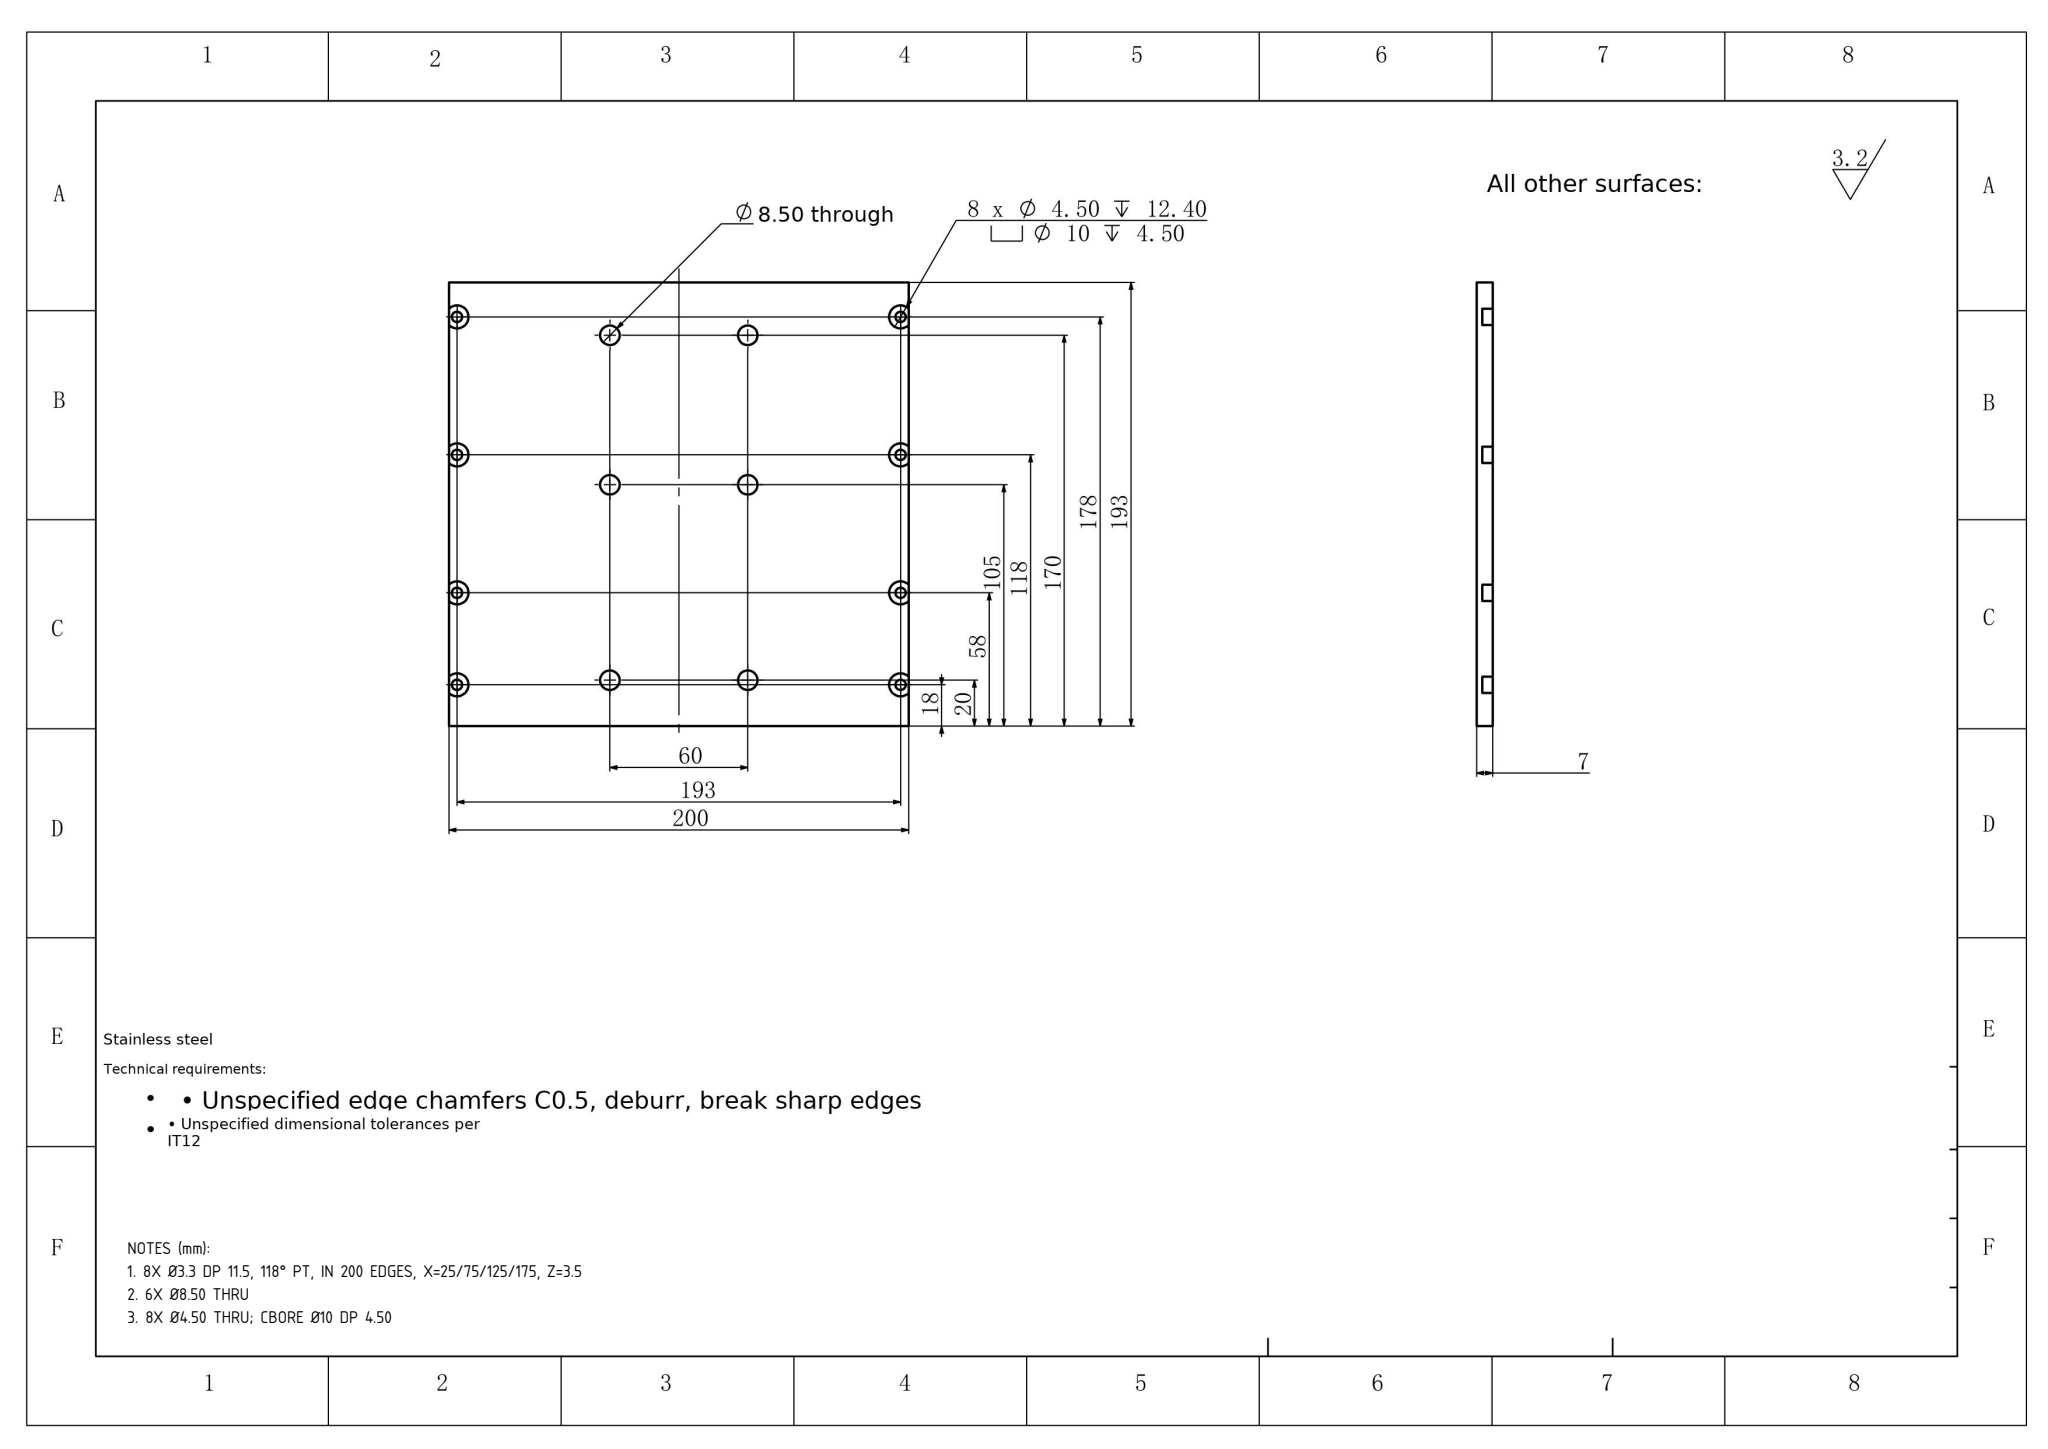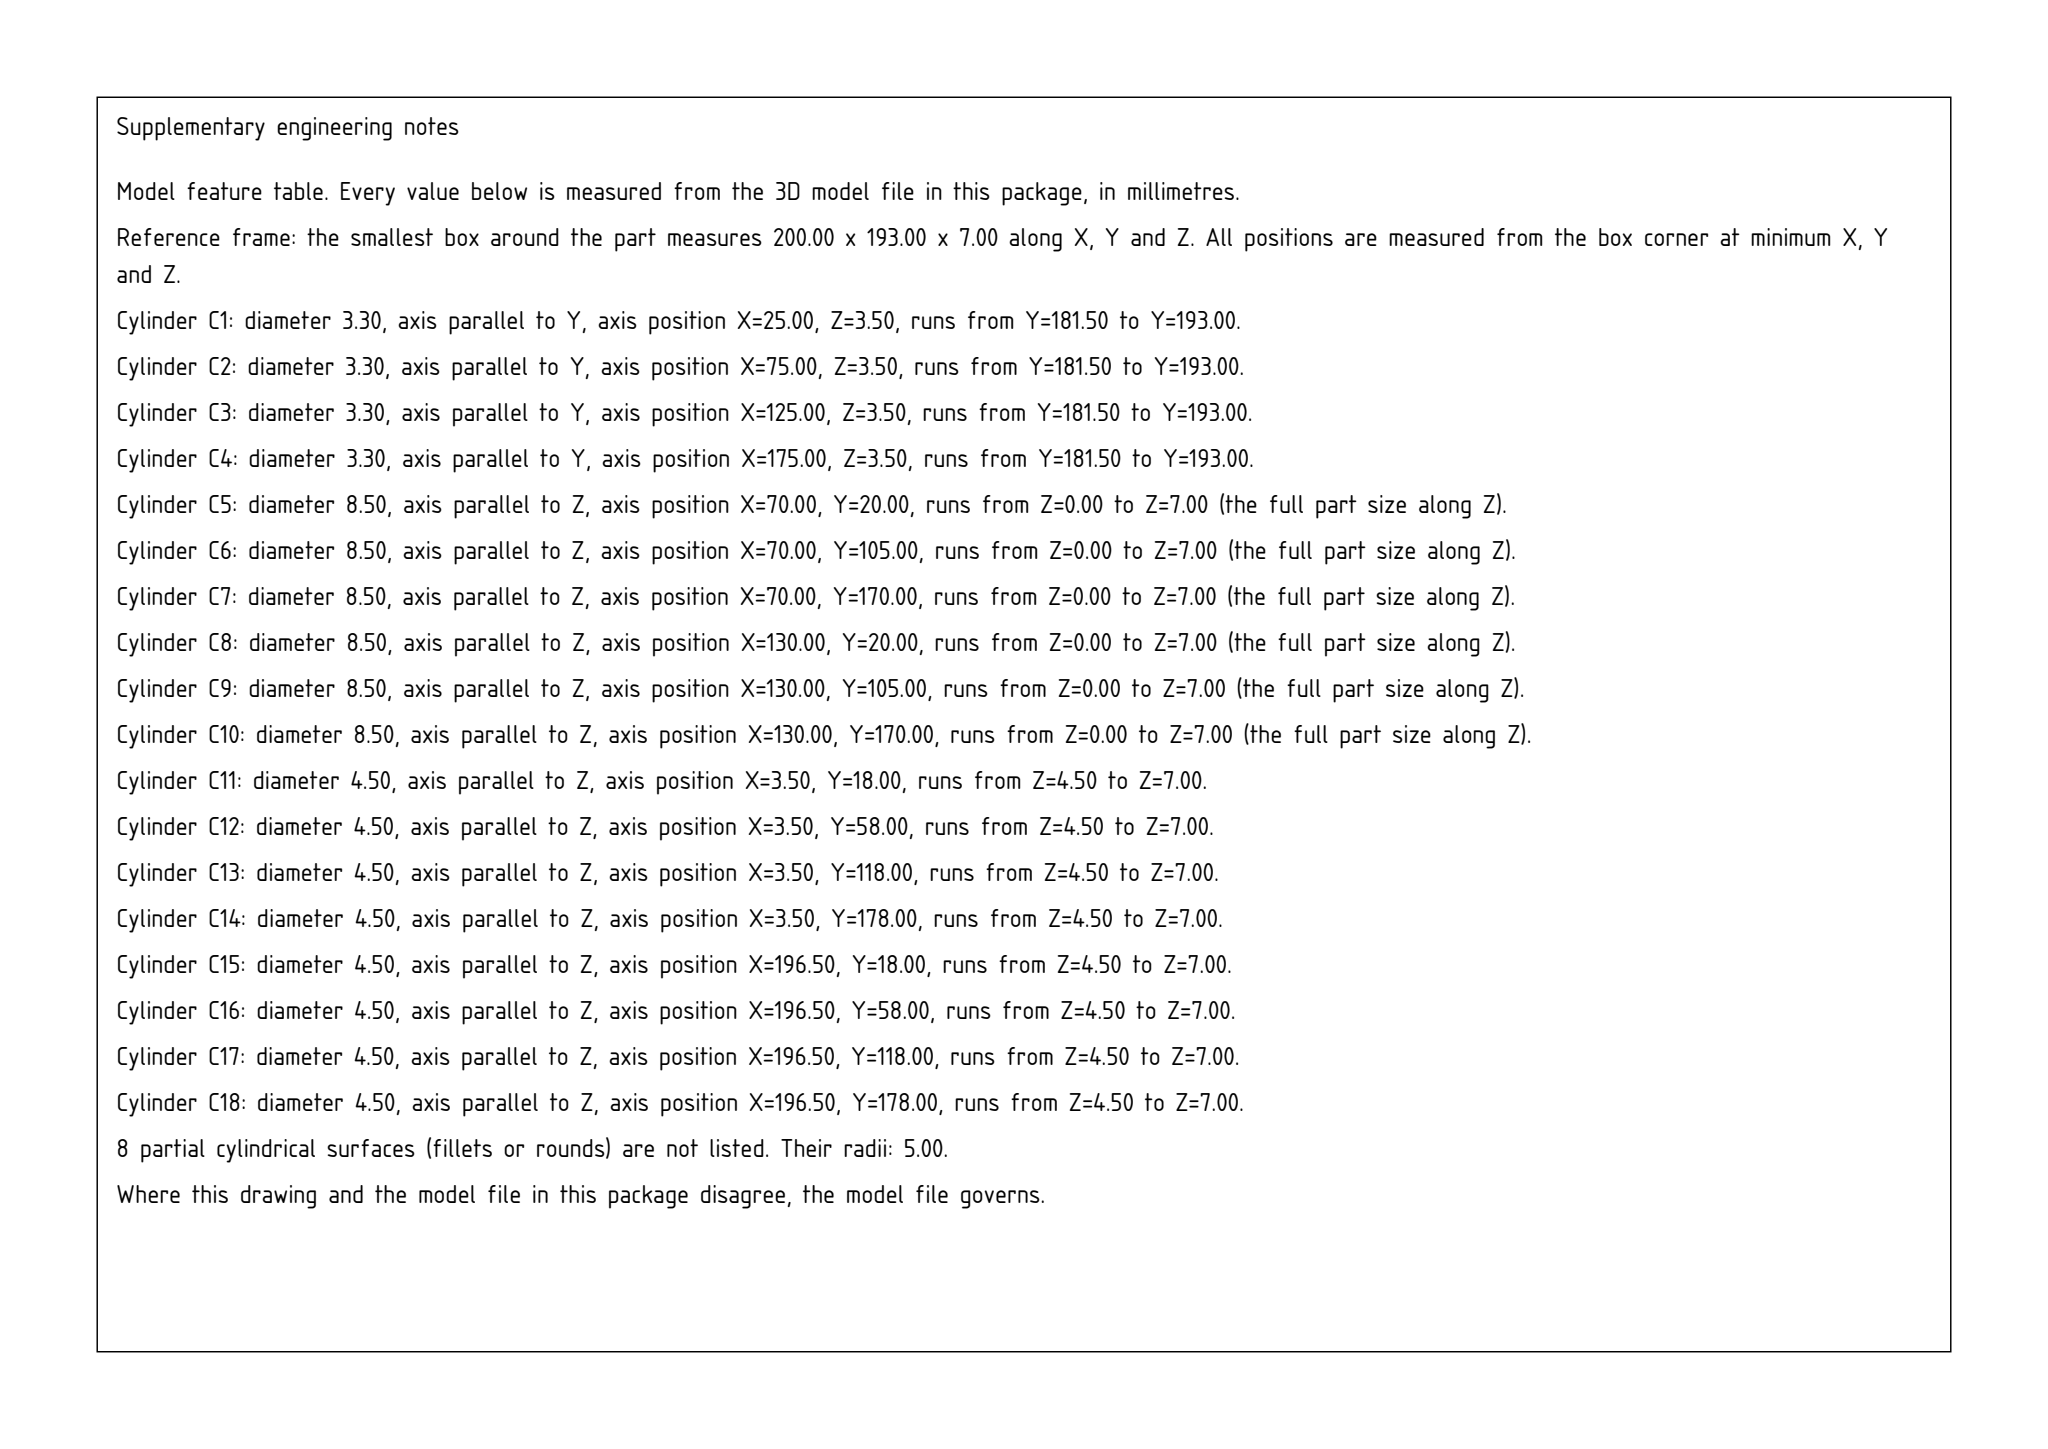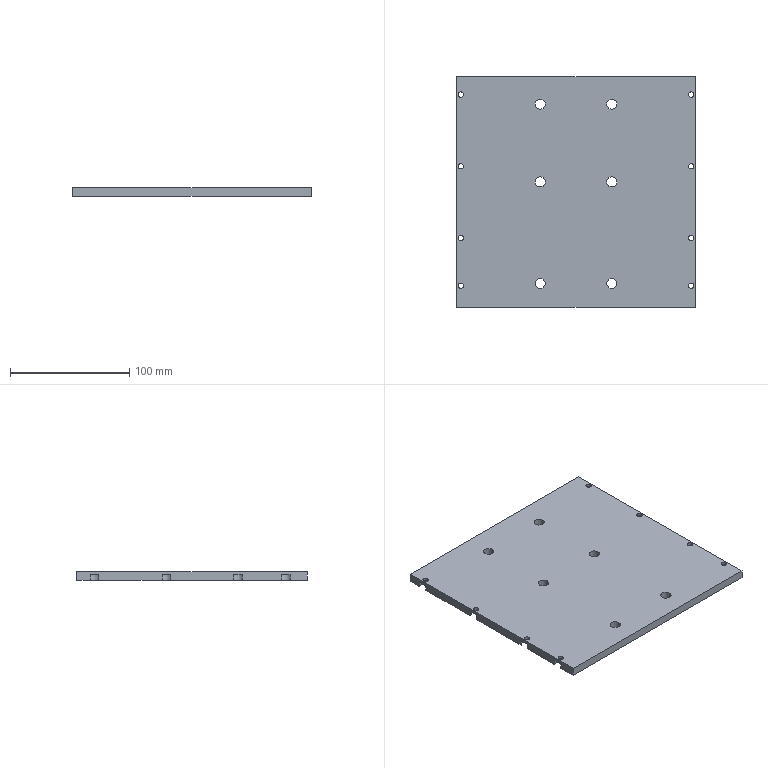Part | SolidWorks | mm | material Stainless steel | 1 solid | 70 faces | box 200 x 193 x 7 mm | volume 264532 mm3 | cylinder 48 | plane 14 | cone 8 | commonest cylinder face diameters 4.5 x16 10 x12 8.5 x12 3.3 x8
Drawing notes:
8X Ø3.3 DP 11.5, 118° PT, IN 200 EDGES, X=25/75/125/175, Z=3.5 | from the solid: cyl dia 3.3 axis y pos [25/75/125/175, -, 3.5] len 11.5 x2 each; cone 118° ref dia 3.3 x8
6X Ø8.50 THRU | from the solid: cyl dia 8.5 axis z at (70/130, 20/105/170) len 7.0 = plate thk
8X Ø4.50 THRU; CBORE Ø10 DP 4.50 | from the solid: cyl dia 4.5 len 2.5 + dia 10 len 4.5 = 7.0 plate thk, 8 locations
build123d program:
from build123d import *

# Parameters (mm, degrees)
SKETCH1_W                                      = 200
SKETCH1_H                                      = 193
BOSS_EXTRUDE1_DEPTH                            = 7
SKETCH2_R                                      = 4.25
CUT_EXTRUDE1_DEPTH                             = 140.145
M4_HEX_HEAD_BOLT_COUNTERBORE_HOLE1_D           = 4.5
M4_HEX_HEAD_BOLT_COUNTERBORE_HOLE1_DEPTH       = 12.4
M4_HEX_HEAD_BOLT_COUNTERBORE_HOLE1_CBORE_D     = 10
M4_HEX_HEAD_BOLT_COUNTERBORE_HOLE1_CBORE_DEPTH = 4.5
M4_HEX_HEAD_BOLT_COUNTERBORE_HOLE1_TIP         = 1.352
M4_TAPPED_HOLE1_D                              = 3.3
M4_TAPPED_HOLE1_DEPTH                          = 11.5
M4_TAPPED_HOLE1_TIP                            = 0.9914


with BuildPart() as part:
    # Sketch1 → Boss-Extrude1 (new body)
    with BuildSketch(Plane.XY):
        Rectangle(SKETCH1_W, SKETCH1_H)
    extrude(amount=BOSS_EXTRUDE1_DEPTH)

    # Sketch2 → Cut-Extrude1 (cut, through all)
    with BuildSketch(Plane.XY.offset(7)):
        with Locations((-30, 73.5)):
            Circle(SKETCH2_R)
        with Locations((-30, 8.5)):
            Circle(SKETCH2_R)
        with Locations((-30, -76.5)):
            Circle(SKETCH2_R)
        with Locations(Location((30, -76.5, 0), (0, 0, 180))):
            Circle(SKETCH2_R)
        with Locations(Location((30, 8.5, 0), (0, 0, 180))):
            Circle(SKETCH2_R)
        with Locations(Location((30, 73.5, 0), (0, 0, 180))):
            Circle(SKETCH2_R)
    extrude(amount=-CUT_EXTRUDE1_DEPTH, mode=Mode.SUBTRACT)

    # M4 Hex Head Bolt Counterbore Hole1
    with Locations(Plane(origin=(0, 0, 0), x_dir=(-1, 0, 0), z_dir=(0, 0, -1))):
        with Locations((96.5, 81.5), (96.5, 21.5), (96.5, -38.5), (-96.5, 81.5), (-96.5, 21.5), (-96.5, -38.5), (-96.5, -78.5), (96.5, -78.5)):
            CounterBoreHole(M4_HEX_HEAD_BOLT_COUNTERBORE_HOLE1_D / 2, M4_HEX_HEAD_BOLT_COUNTERBORE_HOLE1_CBORE_D / 2, M4_HEX_HEAD_BOLT_COUNTERBORE_HOLE1_CBORE_DEPTH, depth=M4_HEX_HEAD_BOLT_COUNTERBORE_HOLE1_DEPTH)
            with Locations((0, 0, -(M4_HEX_HEAD_BOLT_COUNTERBORE_HOLE1_DEPTH + M4_HEX_HEAD_BOLT_COUNTERBORE_HOLE1_TIP / 2))):  # 118° drill point
                Cone(0, M4_HEX_HEAD_BOLT_COUNTERBORE_HOLE1_D / 2, M4_HEX_HEAD_BOLT_COUNTERBORE_HOLE1_TIP, mode=Mode.SUBTRACT)

    # M4 Tapped Hole1
    with Locations(Plane(origin=(0, 96.5, 0), x_dir=(1, 0, 0), z_dir=(0, 1, 0))):
        with Locations((-75, -3.5), (-25, -3.5), (25, -3.5), (75, -3.5)):
            Hole(M4_TAPPED_HOLE1_D / 2, depth=M4_TAPPED_HOLE1_DEPTH)
            with Locations((0, 0, -(M4_TAPPED_HOLE1_DEPTH + M4_TAPPED_HOLE1_TIP / 2))):  # 118° drill point
                Cone(0, M4_TAPPED_HOLE1_D / 2, M4_TAPPED_HOLE1_TIP, mode=Mode.SUBTRACT)


solid = part.part